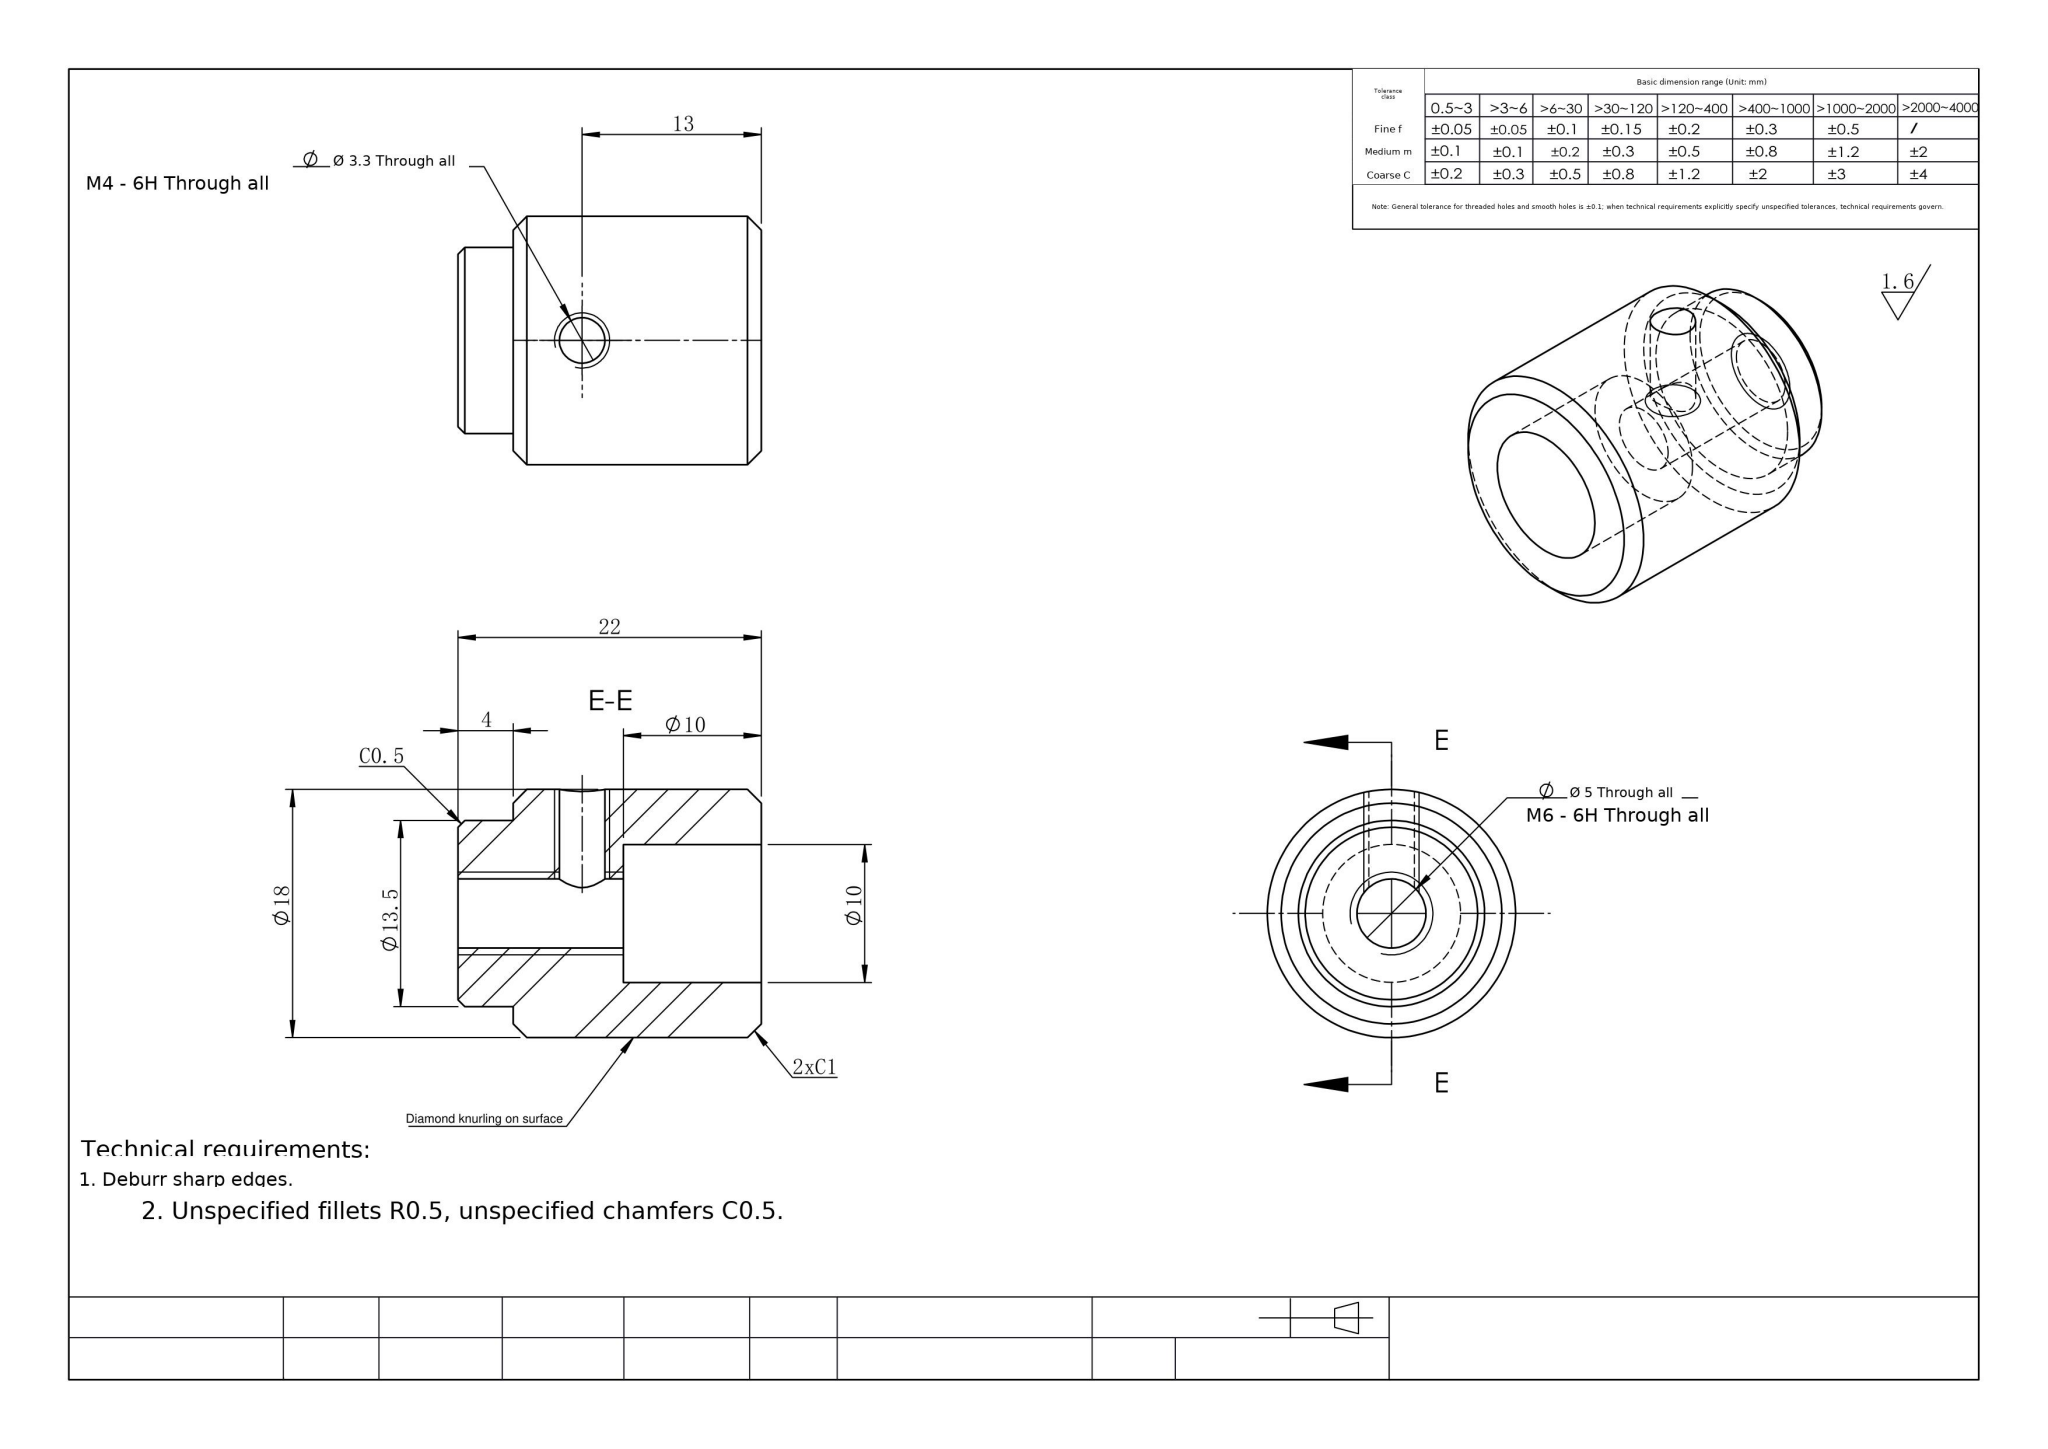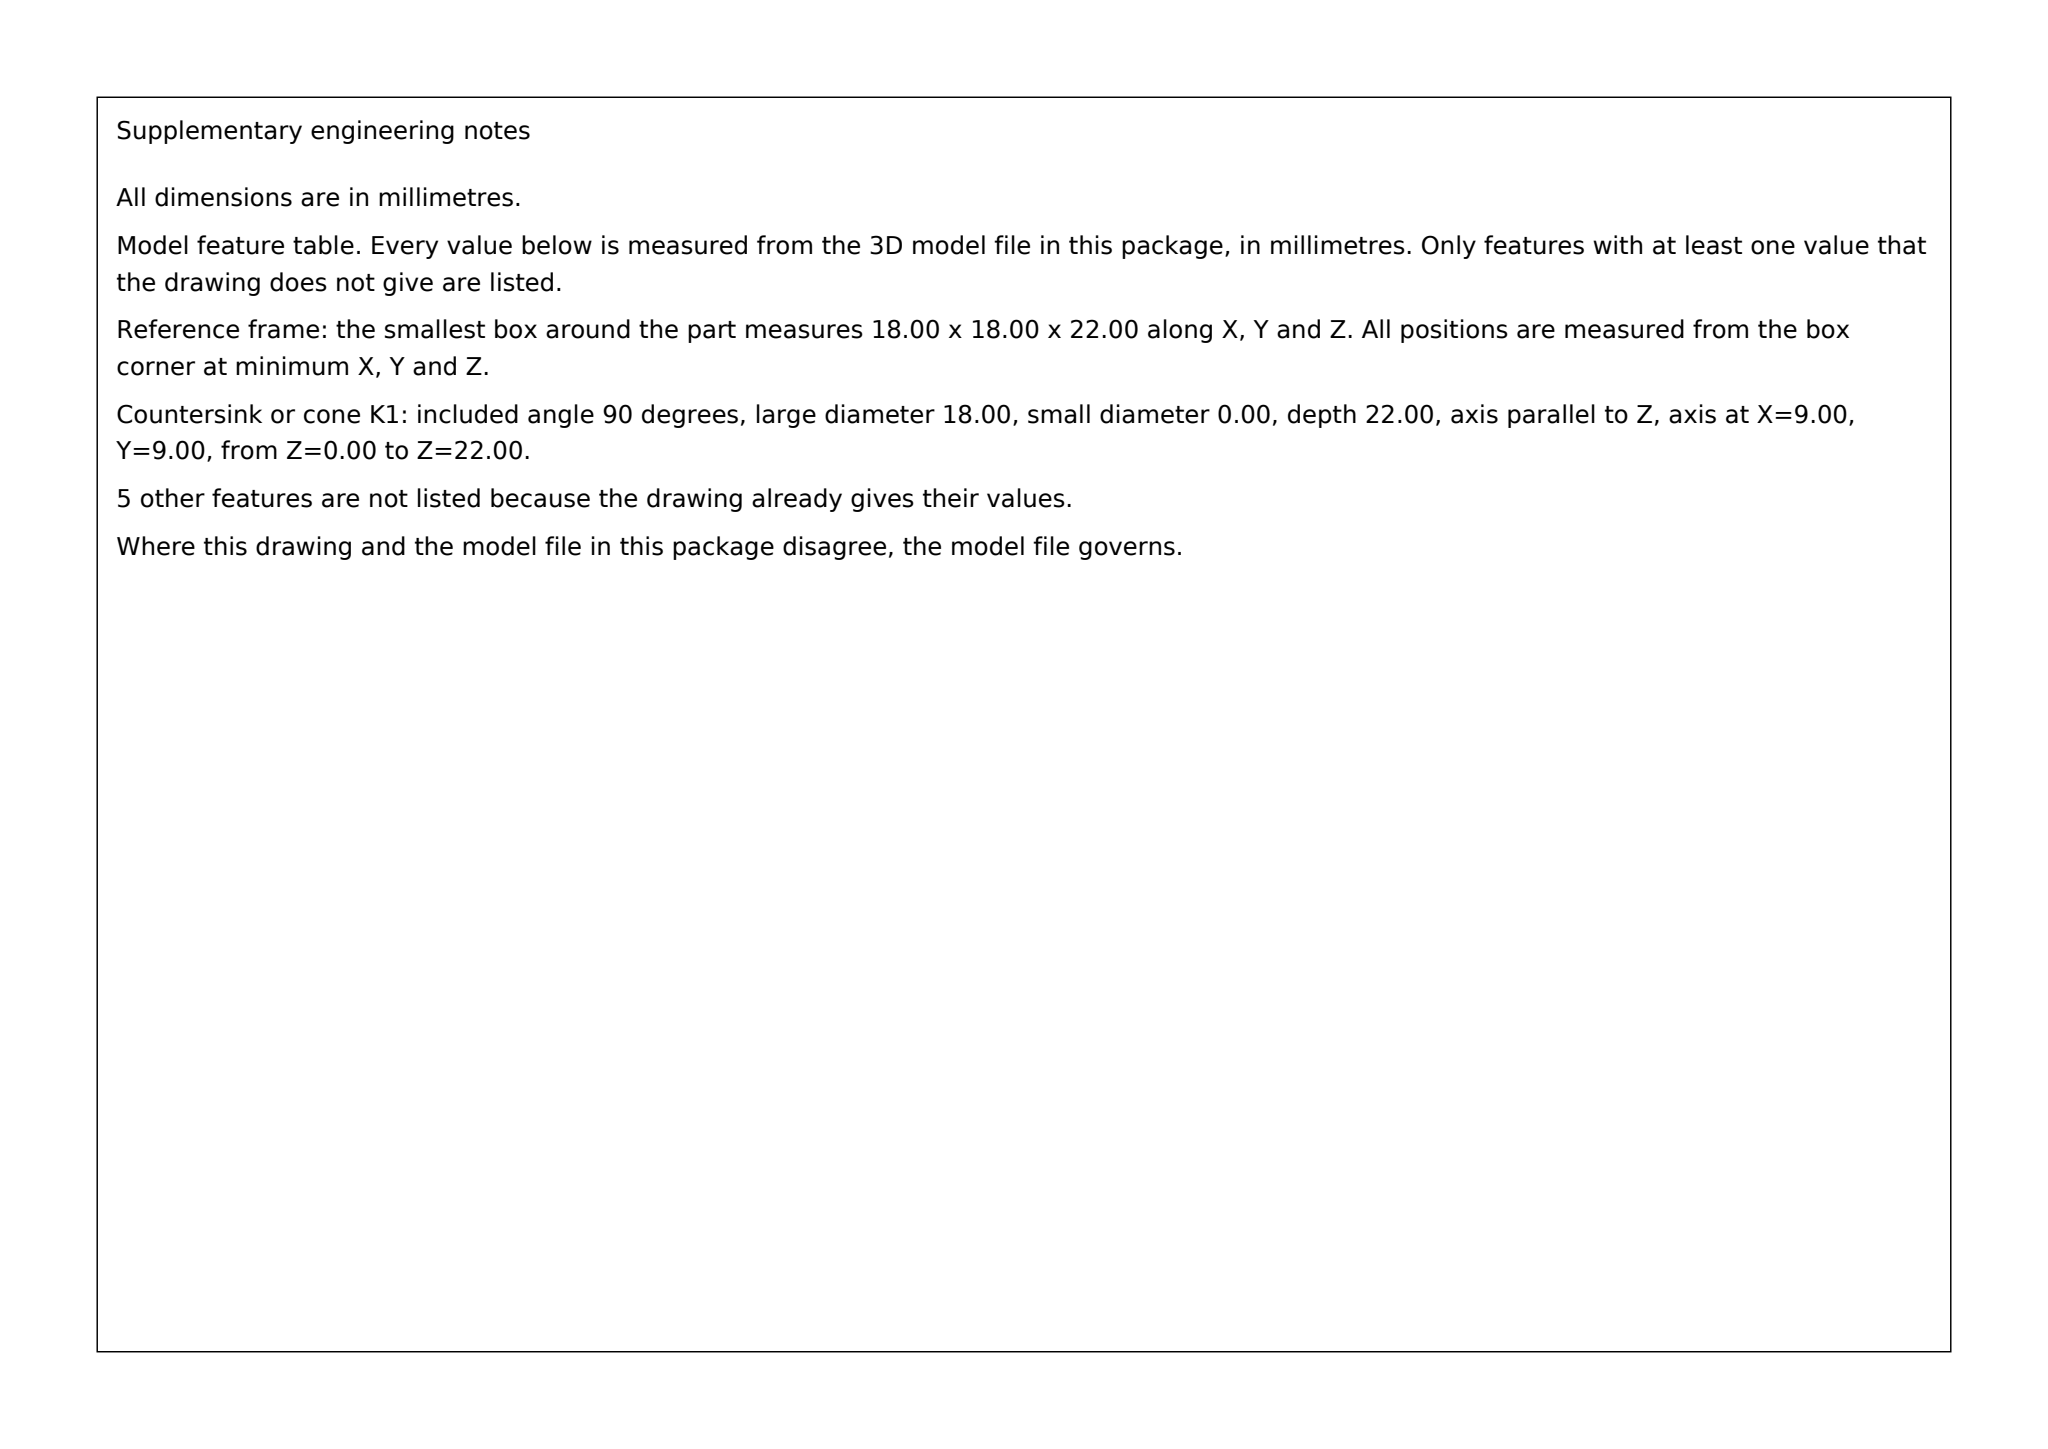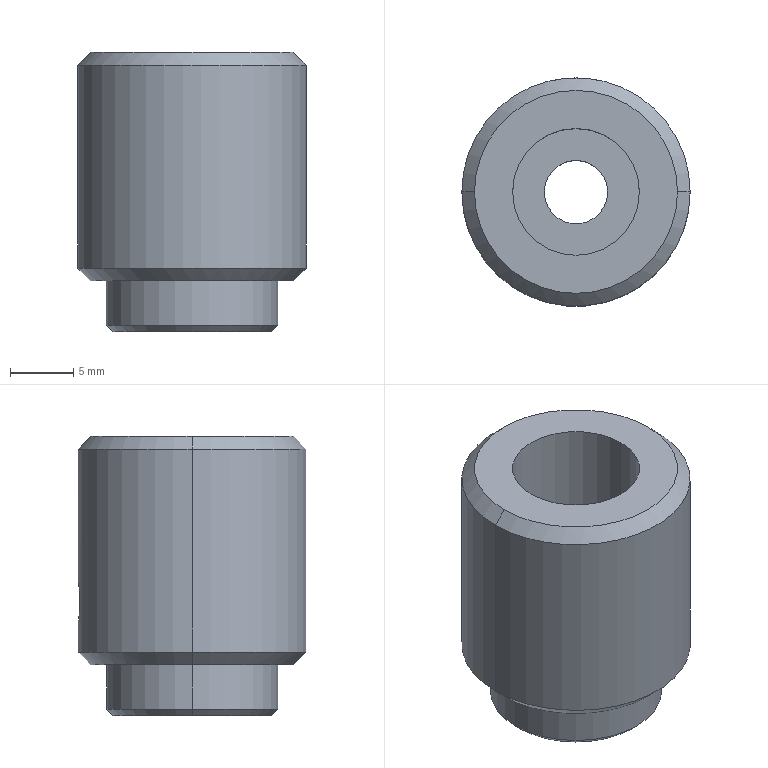Part | SolidWorks | mm | 1 solid | 20 faces | box 18 x 18 x 22 mm | volume 4016 mm3 | cylinder 10 | cone 6 | plane 4 | commonest cylinder face diameters 3.3 x2 5 x2 13.5 x2 10 x2 18 x2
build123d program:
from build123d import *

# Parameters (mm, degrees)
SKETCH1_R           = 9
BOSS_EXTRUDE1_DEPTH = 18
CHAMFER1_SIZE       = 1
SKETCH4_R           = 5
CUT_EXTRUDE1_DEPTH  = 10
SKETCH5_R           = 6.75
BOSS_EXTRUDE2_DEPTH = 4
M6_TAPPED_HOLE2_D   = 5
CHAMFER2_SIZE       = 0.5
SKETCH9_W           = 1.65
SKETCH9_H           = 9


with BuildPart() as part:
    # Sketch1 → Boss-Extrude1 (new body)
    with BuildSketch(Plane.XY):
        Circle(SKETCH1_R)
    extrude(amount=BOSS_EXTRUDE1_DEPTH)

    # Chamfer1
    chamfer1_edges = [part.edges().sort_by_distance(p)[0] for p in [
        (-9, 0, 0),
        (-9, 0, 18),
    ]]
    chamfer(chamfer1_edges, length=CHAMFER1_SIZE)

    # Sketch4 → Cut-Extrude1 (cut)
    with BuildSketch(Plane.XY.offset(18)):
        Circle(SKETCH4_R)
    extrude(amount=-CUT_EXTRUDE1_DEPTH, mode=Mode.SUBTRACT)

    # Sketch5 → Boss-Extrude2 (add)
    with BuildSketch(Plane(origin=(0, 0, 0), x_dir=(-1, 0, 0), z_dir=(0, 0, -1))):
        with Locations(Location((0, 0, 0), (0, 0, 180))):
            Circle(SKETCH5_R)
    extrude(amount=BOSS_EXTRUDE2_DEPTH)

    # M6 Tapped Hole2 (through all)
    with Locations(Plane(origin=(0, 0, -4), x_dir=(-1, 0, 0), z_dir=(0, 0, -1))):
        with Locations((0, 0)):
            Hole(M6_TAPPED_HOLE2_D / 2)

    # Chamfer2
    chamfer2_edges = [part.edges().sort_by_distance(p)[0] for p in [
        (-6.75, 0, -4),
    ]]
    chamfer(chamfer2_edges, length=CHAMFER2_SIZE)

    # Sketch9 → M4 Tapped Hole1 (revolve, cut)
    with BuildSketch(Plane(origin=(0, 0, 5), x_dir=(0, 0, -1), z_dir=(1, 0, 0))):
        with Locations((0.825, 4.5)):
            Rectangle(SKETCH9_W, SKETCH9_H)
    revolve(axis=Axis((0, -6.35, 5), (0, 1, 0)), mode=Mode.SUBTRACT)


solid = part.part
STEP:
#1=CARTESIAN_POINT('',(0.,9.,6.65));
#2=VERTEX_POINT('',#1);
#3=CARTESIAN_POINT('',(0.,9.,3.35));
#4=VERTEX_POINT('',#3);
#5=CARTESIAN_POINT('',(0.,9.,6.65));
#6=CARTESIAN_POINT('',(-0.2156,9.,6.65));
#7=CARTESIAN_POINT('',(-0.4331,8.992,6.607));
#8=CARTESIAN_POINT('',(-0.8303,8.964,6.442));
#9=CARTESIAN_POINT('',(-1.014,8.944,6.319));
#10=CARTESIAN_POINT('',(-1.242,8.914,6.091));
#11=CARTESIAN_POINT('',(-1.312,8.904,6.007));
#12=CARTESIAN_POINT('',(-1.431,8.886,5.828));
#13=CARTESIAN_POINT('',(-1.482,8.877,5.733));
#14=CARTESIAN_POINT('',(-1.607,8.856,5.433));
#15=CARTESIAN_POINT('',(-1.65,8.847,5.219));
#16=CARTESIAN_POINT('',(-1.65,8.847,4.892));
#17=CARTESIAN_POINT('',(-1.639,8.849,4.785));
#18=CARTESIAN_POINT('',(-1.598,8.857,4.573));
#19=CARTESIAN_POINT('',(-1.566,8.863,4.468));
#20=CARTESIAN_POINT('',(-1.483,8.877,4.269));
#21=CARTESIAN_POINT('',(-1.432,8.885,4.174));
#22=CARTESIAN_POINT('',(-1.313,8.904,3.994));
#23=CARTESIAN_POINT('',(-1.243,8.914,3.91));
#24=CARTESIAN_POINT('',(-1.016,8.944,3.682));
#25=CARTESIAN_POINT('',(-0.8322,8.964,3.559));
#26=CARTESIAN_POINT('',(-0.4354,8.992,3.394));
#27=CARTESIAN_POINT('',(-0.2185,9.,3.35));
#28=CARTESIAN_POINT('',(0.,9.,3.35));
#29=B_SPLINE_CURVE_WITH_KNOTS('',3,(#5,#6,#7,#8,#9,#10,#11,#12,#13,#14,#15,#16,#17,#18,#19,#20,#21,#22,#23,#24,#25,#26,#27,#28),.UNSPECIFIED.,.F.,.F.,(4,2,2,2,2,2,2,2,2,2,2,4),(0.00517,0.005816,0.006462,0.006785,0.007108,0.007754,0.008077,0.0084,0.008723,0.009046,0.009692,0.01034),.UNSPECIFIED.);
#30=EDGE_CURVE('',#2,#4,#29,.T.);
#31=ORIENTED_EDGE('',*,*,#30,.F.);
#32=CARTESIAN_POINT('',(0.,2.5,6.65));
#33=VERTEX_POINT('',#32);
#34=CARTESIAN_POINT('',(0.,0.,6.65));
#35=DIRECTION('',(0.,-1.,0.));
#36=VECTOR('',#35,1000.);
#37=LINE('',#34,#36);
#38=EDGE_CURVE('',#2,#33,#37,.T.);
#39=ORIENTED_EDGE('',*,*,#38,.T.);
#40=CARTESIAN_POINT('',(0.,2.5,3.35));
#41=VERTEX_POINT('',#40);
#42=CARTESIAN_POINT('',(0.,2.5,3.35));
#43=CARTESIAN_POINT('',(-0.1128,2.5,3.35));
#44=CARTESIAN_POINT('',(-0.2231,2.492,3.361));
#45=CARTESIAN_POINT('',(-0.4392,2.464,3.406));
#46=CARTESIAN_POINT('',(-0.5457,2.442,3.439));
#47=CARTESIAN_POINT('',(-0.8444,2.362,3.566));
#48=CARTESIAN_POINT('',(-1.022,2.287,3.688));
#49=CARTESIAN_POINT('',(-1.243,2.171,3.91));
#50=CARTESIAN_POINT('',(-1.31,2.13,3.992));
#51=CARTESIAN_POINT('',(-1.427,2.054,4.165));
#52=CARTESIAN_POINT('',(-1.477,2.017,4.257));
#53=CARTESIAN_POINT('',(-1.602,1.922,4.552));
#54=CARTESIAN_POINT('',(-1.65,1.878,4.775));
#55=CARTESIAN_POINT('',(-1.65,1.878,5.222));
#56=CARTESIAN_POINT('',(-1.604,1.921,5.443));
#57=CARTESIAN_POINT('',(-1.437,2.048,5.839));
#58=CARTESIAN_POINT('',(-1.318,2.131,6.015));
#59=CARTESIAN_POINT('',(-1.096,2.249,6.238));
#60=CARTESIAN_POINT('',(-1.015,2.287,6.305));
#61=CARTESIAN_POINT('',(-0.8408,2.356,6.424));
#62=CARTESIAN_POINT('',(-0.7457,2.388,6.476));
#63=CARTESIAN_POINT('',(-0.5456,2.442,6.561));
#64=CARTESIAN_POINT('',(-0.4413,2.463,6.594));
#65=CARTESIAN_POINT('',(-0.2236,2.492,6.639));
#66=CARTESIAN_POINT('',(-0.1111,2.5,6.65));
#67=CARTESIAN_POINT('',(0.,2.5,6.65));
#68=B_SPLINE_CURVE_WITH_KNOTS('',3,(#42,#43,#44,#45,#46,#47,#48,#49,#50,#51,#52,#53,#54,#55,#56,#57,#58,#59,#60,#61,#62,#63,#64,#65,#66,#67),.UNSPECIFIED.,.F.,.F.,(4,2,2,2,2,2,2,2,2,2,2,2,4),(0.,0.000333,0.000666,0.001332,0.001665,0.001998,0.002664,0.00333,0.003996,0.004329,0.004662,0.004995,0.005328),.UNSPECIFIED.);
#69=EDGE_CURVE('',#41,#33,#68,.T.);
#70=ORIENTED_EDGE('',*,*,#69,.F.);
#71=CARTESIAN_POINT('',(0.,0.,3.35));
#72=DIRECTION('',(0.,-1.,0.));
#73=VECTOR('',#72,1000.);
#74=LINE('',#71,#73);
#75=EDGE_CURVE('',#4,#41,#74,.T.);
#76=ORIENTED_EDGE('',*,*,#75,.F.);
#77=EDGE_LOOP('',(#31,#39,#70,#76));
#78=FACE_OUTER_BOUND('',#77,.T.);
#79=CARTESIAN_POINT('',(0.,0.,5.));
#80=DIRECTION('',(0.,-1.,0.));
#81=DIRECTION('',(0.,0.,-1.));
#82=AXIS2_PLACEMENT_3D('',#79,#80,#81);
#83=CYLINDRICAL_SURFACE('',#82,1.65);
#84=ADVANCED_FACE('',(#78),#83,.F.);
#85=CARTESIAN_POINT('',(-6.25,0.,-4.));
#86=VERTEX_POINT('',#85);
#87=CARTESIAN_POINT('',(6.25,0.,-4.));
#88=VERTEX_POINT('',#87);
#89=CARTESIAN_POINT('',(0.,0.,-4.));
#90=DIRECTION('',(0.,0.,-1.));
#91=DIRECTION('',(-1.,0.,0.));
#92=AXIS2_PLACEMENT_3D('',#89,#90,#91);
#93=CIRCLE('',#92,6.25);
#94=EDGE_CURVE('',#86,#88,#93,.T.);
#95=ORIENTED_EDGE('',*,*,#94,.F.);
#96=CARTESIAN_POINT('',(-6.75,0.,-3.5));
#97=VERTEX_POINT('',#96);
#98=CARTESIAN_POINT('',(-6.25,0.,-4.));
#99=DIRECTION('',(-0.7071,0.,0.7071));
#100=VECTOR('',#99,1000.);
#101=LINE('',#98,#100);
#102=EDGE_CURVE('',#86,#97,#101,.T.);
#103=ORIENTED_EDGE('',*,*,#102,.T.);
#104=CARTESIAN_POINT('',(6.75,0.,-3.5));
#105=VERTEX_POINT('',#104);
#106=CARTESIAN_POINT('',(0.,0.,-3.5));
#107=DIRECTION('',(0.,0.,1.));
#108=DIRECTION('',(-1.,0.,0.));
#109=AXIS2_PLACEMENT_3D('',#106,#107,#108);
#110=CIRCLE('',#109,6.75);
#111=EDGE_CURVE('',#105,#97,#110,.T.);
#112=ORIENTED_EDGE('',*,*,#111,.F.);
#113=CARTESIAN_POINT('',(6.25,0.,-4.));
#114=DIRECTION('',(0.7071,0.,0.7071));
#115=VECTOR('',#114,1000.);
#116=LINE('',#113,#115);
#117=EDGE_CURVE('',#88,#105,#116,.T.);
#118=ORIENTED_EDGE('',*,*,#117,.F.);
#119=EDGE_LOOP('',(#95,#103,#112,#118));
#120=FACE_OUTER_BOUND('',#119,.T.);
#121=CARTESIAN_POINT('',(0.,0.,-4.));
#122=DIRECTION('',(0.,0.,1.));
#123=DIRECTION('',(1.,0.,0.));
#124=AXIS2_PLACEMENT_3D('',#121,#122,#123);
#125=CONICAL_SURFACE('',#124,6.25,0.7854);
#126=ADVANCED_FACE('',(#120),#125,.T.);
#127=CARTESIAN_POINT('',(-2.5,0.,8.));
#128=VERTEX_POINT('',#127);
#129=CARTESIAN_POINT('',(2.5,0.,8.));
#130=VERTEX_POINT('',#129);
#131=CARTESIAN_POINT('',(0.,0.,8.));
#132=DIRECTION('',(0.,0.,1.));
#133=DIRECTION('',(1.,0.,0.));
#134=AXIS2_PLACEMENT_3D('',#131,#132,#133);
#135=CIRCLE('',#134,2.5);
#136=EDGE_CURVE('',#128,#130,#135,.T.);
#137=ORIENTED_EDGE('',*,*,#136,.T.);
#138=CARTESIAN_POINT('',(2.5,0.,-4.));
#139=VERTEX_POINT('',#138);
#140=CARTESIAN_POINT('',(2.5,0.,-4.));
#141=DIRECTION('',(0.,0.,-1.));
#142=VECTOR('',#141,1000.);
#143=LINE('',#140,#142);
#144=EDGE_CURVE('',#130,#139,#143,.T.);
#145=ORIENTED_EDGE('',*,*,#144,.T.);
#146=CARTESIAN_POINT('',(-2.5,0.,-4.));
#147=VERTEX_POINT('',#146);
#148=CARTESIAN_POINT('',(0.,0.,-4.));
#149=DIRECTION('',(0.,0.,-1.));
#150=DIRECTION('',(-1.,0.,0.));
#151=AXIS2_PLACEMENT_3D('',#148,#149,#150);
#152=CIRCLE('',#151,2.5);
#153=EDGE_CURVE('',#139,#147,#152,.T.);
#154=ORIENTED_EDGE('',*,*,#153,.T.);
#155=CARTESIAN_POINT('',(-2.5,0.,-4.));
#156=DIRECTION('',(0.,0.,-1.));
#157=VECTOR('',#156,1000.);
#158=LINE('',#155,#157);
#159=EDGE_CURVE('',#128,#147,#158,.T.);
#160=ORIENTED_EDGE('',*,*,#159,.F.);
#161=EDGE_LOOP('',(#137,#145,#154,#160));
#162=FACE_OUTER_BOUND('',#161,.T.);
#163=CARTESIAN_POINT('',(0.,0.,-4.));
#164=DIRECTION('',(0.,0.,-1.));
#165=DIRECTION('',(-1.,0.,0.));
#166=AXIS2_PLACEMENT_3D('',#163,#164,#165);
#167=CYLINDRICAL_SURFACE('',#166,2.5);
#168=ADVANCED_FACE('',(#162),#167,.F.);
#169=ORIENTED_EDGE('',*,*,#111,.T.);
#170=CARTESIAN_POINT('',(-6.75,0.,0.));
#171=VERTEX_POINT('',#170);
#172=CARTESIAN_POINT('',(-6.75,0.,-4.));
#173=DIRECTION('',(0.,0.,1.));
#174=VECTOR('',#173,1000.);
#175=LINE('',#172,#174);
#176=EDGE_CURVE('',#97,#171,#175,.T.);
#177=ORIENTED_EDGE('',*,*,#176,.T.);
#178=CARTESIAN_POINT('',(6.75,0.,0.));
#179=VERTEX_POINT('',#178);
#180=CARTESIAN_POINT('',(0.,0.,0.));
#181=DIRECTION('',(0.,0.,-1.));
#182=DIRECTION('',(1.,0.,0.));
#183=AXIS2_PLACEMENT_3D('',#180,#181,#182);
#184=CIRCLE('',#183,6.75);
#185=EDGE_CURVE('',#171,#179,#184,.T.);
#186=ORIENTED_EDGE('',*,*,#185,.T.);
#187=CARTESIAN_POINT('',(6.75,0.,-4.));
#188=DIRECTION('',(0.,0.,1.));
#189=VECTOR('',#188,1000.);
#190=LINE('',#187,#189);
#191=EDGE_CURVE('',#105,#179,#190,.T.);
#192=ORIENTED_EDGE('',*,*,#191,.F.);
#193=EDGE_LOOP('',(#169,#177,#186,#192));
#194=FACE_OUTER_BOUND('',#193,.T.);
#195=CARTESIAN_POINT('',(0.,0.,-4.));
#196=DIRECTION('',(0.,0.,1.));
#197=DIRECTION('',(1.,0.,0.));
#198=AXIS2_PLACEMENT_3D('',#195,#196,#197);
#199=CYLINDRICAL_SURFACE('',#198,6.75);
#200=ADVANCED_FACE('',(#194),#199,.T.);
#201=CARTESIAN_POINT('',(-5.,0.,8.));
#202=VERTEX_POINT('',#201);
#203=CARTESIAN_POINT('',(5.,0.,8.));
#204=VERTEX_POINT('',#203);
#205=CARTESIAN_POINT('',(0.,0.,8.));
#206=DIRECTION('',(0.,0.,1.));
#207=DIRECTION('',(1.,0.,0.));
#208=AXIS2_PLACEMENT_3D('',#205,#206,#207);
#209=CIRCLE('',#208,5.);
#210=EDGE_CURVE('',#202,#204,#209,.T.);
#211=ORIENTED_EDGE('',*,*,#210,.F.);
#212=CARTESIAN_POINT('',(-5.,0.,18.));
#213=VERTEX_POINT('',#212);
#214=CARTESIAN_POINT('',(-5.,0.,8.));
#215=DIRECTION('',(0.,0.,1.));
#216=VECTOR('',#215,1000.);
#217=LINE('',#214,#216);
#218=EDGE_CURVE('',#202,#213,#217,.T.);
#219=ORIENTED_EDGE('',*,*,#218,.T.);
#220=CARTESIAN_POINT('',(5.,0.,18.));
#221=VERTEX_POINT('',#220);
#222=CARTESIAN_POINT('',(0.,0.,18.));
#223=DIRECTION('',(0.,0.,1.));
#224=DIRECTION('',(1.,0.,0.));
#225=AXIS2_PLACEMENT_3D('',#222,#223,#224);
#226=CIRCLE('',#225,5.);
#227=EDGE_CURVE('',#213,#221,#226,.T.);
#228=ORIENTED_EDGE('',*,*,#227,.T.);
#229=CARTESIAN_POINT('',(5.,0.,8.));
#230=DIRECTION('',(0.,0.,1.));
#231=VECTOR('',#230,1000.);
#232=LINE('',#229,#231);
#233=EDGE_CURVE('',#204,#221,#232,.T.);
#234=ORIENTED_EDGE('',*,*,#233,.F.);
#235=EDGE_LOOP('',(#211,#219,#228,#234));
#236=FACE_OUTER_BOUND('',#235,.T.);
#237=CARTESIAN_POINT('',(0.,0.,8.));
#238=DIRECTION('',(0.,0.,1.));
#239=DIRECTION('',(1.,0.,0.));
#240=AXIS2_PLACEMENT_3D('',#237,#238,#239);
#241=CYLINDRICAL_SURFACE('',#240,5.);
#242=ADVANCED_FACE('',(#236),#241,.F.);
#243=CARTESIAN_POINT('',(-8.,0.,0.));
#244=VERTEX_POINT('',#243);
#245=CARTESIAN_POINT('',(8.,0.,0.));
#246=VERTEX_POINT('',#245);
#247=CARTESIAN_POINT('',(0.,0.,0.));
#248=DIRECTION('',(0.,0.,-1.));
#249=DIRECTION('',(1.,0.,0.));
#250=AXIS2_PLACEMENT_3D('',#247,#248,#249);
#251=CIRCLE('',#250,8.);
#252=EDGE_CURVE('',#244,#246,#251,.T.);
#253=ORIENTED_EDGE('',*,*,#252,.F.);
#254=CARTESIAN_POINT('',(-9.,0.,1.));
#255=VERTEX_POINT('',#254);
#256=CARTESIAN_POINT('',(-9.,0.,1.));
#257=DIRECTION('',(-0.7071,0.,0.7071));
#258=VECTOR('',#257,1000.);
#259=LINE('',#256,#258);
#260=EDGE_CURVE('',#244,#255,#259,.T.);
#261=ORIENTED_EDGE('',*,*,#260,.T.);
#262=CARTESIAN_POINT('',(9.,0.,1.));
#263=VERTEX_POINT('',#262);
#264=CARTESIAN_POINT('',(0.,0.,1.));
#265=DIRECTION('',(0.,0.,1.));
#266=DIRECTION('',(1.,0.,0.));
#267=AXIS2_PLACEMENT_3D('',#264,#265,#266);
#268=CIRCLE('',#267,9.);
#269=EDGE_CURVE('',#263,#255,#268,.T.);
#270=ORIENTED_EDGE('',*,*,#269,.F.);
#271=CARTESIAN_POINT('',(9.,0.,1.));
#272=DIRECTION('',(0.7071,0.,0.7071));
#273=VECTOR('',#272,1000.);
#274=LINE('',#271,#273);
#275=EDGE_CURVE('',#246,#263,#274,.T.);
#276=ORIENTED_EDGE('',*,*,#275,.F.);
#277=EDGE_LOOP('',(#253,#261,#270,#276));
#278=FACE_OUTER_BOUND('',#277,.T.);
#279=CARTESIAN_POINT('',(0.,0.,1.));
#280=DIRECTION('',(0.,0.,1.));
#281=DIRECTION('',(1.,0.,0.));
#282=AXIS2_PLACEMENT_3D('',#279,#280,#281);
#283=CONICAL_SURFACE('',#282,9.,0.7854);
#284=ADVANCED_FACE('',(#278),#283,.T.);
#285=CARTESIAN_POINT('',(8.,0.,18.));
#286=VERTEX_POINT('',#285);
#287=CARTESIAN_POINT('',(-8.,0.,18.));
#288=VERTEX_POINT('',#287);
#289=CARTESIAN_POINT('',(0.,0.,18.));
#290=DIRECTION('',(0.,0.,1.));
#291=DIRECTION('',(1.,0.,0.));
#292=AXIS2_PLACEMENT_3D('',#289,#290,#291);
#293=CIRCLE('',#292,8.);
#294=EDGE_CURVE('',#286,#288,#293,.T.);
#295=ORIENTED_EDGE('',*,*,#294,.F.);
#296=CARTESIAN_POINT('',(9.,0.,17.));
#297=VERTEX_POINT('',#296);
#298=CARTESIAN_POINT('',(8.,0.,18.));
#299=DIRECTION('',(0.7071,0.,-0.7071));
#300=VECTOR('',#299,1000.);
#301=LINE('',#298,#300);
#302=EDGE_CURVE('',#286,#297,#301,.T.);
#303=ORIENTED_EDGE('',*,*,#302,.T.);
#304=CARTESIAN_POINT('',(-9.,0.,17.));
#305=VERTEX_POINT('',#304);
#306=CARTESIAN_POINT('',(0.,0.,17.));
#307=DIRECTION('',(0.,0.,-1.));
#308=DIRECTION('',(1.,0.,0.));
#309=AXIS2_PLACEMENT_3D('',#306,#307,#308);
#310=CIRCLE('',#309,9.);
#311=EDGE_CURVE('',#305,#297,#310,.T.);
#312=ORIENTED_EDGE('',*,*,#311,.F.);
#313=CARTESIAN_POINT('',(-8.,0.,18.));
#314=DIRECTION('',(-0.7071,0.,-0.7071));
#315=VECTOR('',#314,1000.);
#316=LINE('',#313,#315);
#317=EDGE_CURVE('',#288,#305,#316,.T.);
#318=ORIENTED_EDGE('',*,*,#317,.F.);
#319=EDGE_LOOP('',(#295,#303,#312,#318));
#320=FACE_OUTER_BOUND('',#319,.T.);
#321=CARTESIAN_POINT('',(0.,0.,18.));
#322=DIRECTION('',(0.,0.,-1.));
#323=DIRECTION('',(-1.,0.,0.));
#324=AXIS2_PLACEMENT_3D('',#321,#322,#323);
#325=CONICAL_SURFACE('',#324,8.,0.7854);
#326=ADVANCED_FACE('',(#320),#325,.T.);
#327=CARTESIAN_POINT('',(0.,9.,3.35));
#328=CARTESIAN_POINT('',(0.1093,9.,3.35));
#329=CARTESIAN_POINT('',(0.2167,8.998,3.361));
#330=CARTESIAN_POINT('',(0.4279,8.99,3.403));
#331=CARTESIAN_POINT('',(0.5328,8.985,3.435));
#332=CARTESIAN_POINT('',(0.7325,8.971,3.518));
#333=CARTESIAN_POINT('',(0.8272,8.962,3.568));
#334=CARTESIAN_POINT('',(1.006,8.944,3.688));
#335=CARTESIAN_POINT('',(1.091,8.934,3.758));
#336=CARTESIAN_POINT('',(1.319,8.904,3.985));
#337=CARTESIAN_POINT('',(1.442,8.884,4.169));
#338=CARTESIAN_POINT('',(1.606,8.856,4.566));
#339=CARTESIAN_POINT('',(1.65,8.847,4.784));
#340=CARTESIAN_POINT('',(1.65,8.847,5.107));
#341=CARTESIAN_POINT('',(1.639,8.849,5.217));
#342=CARTESIAN_POINT('',(1.597,8.857,5.429));
#343=CARTESIAN_POINT('',(1.566,8.863,5.532));
#344=CARTESIAN_POINT('',(1.441,8.884,5.832));
#345=CARTESIAN_POINT('',(1.32,8.904,6.013));
#346=CARTESIAN_POINT('',(1.09,8.934,6.244));
#347=CARTESIAN_POINT('',(1.007,8.944,6.312));
#348=CARTESIAN_POINT('',(0.8283,8.962,6.431));
#349=CARTESIAN_POINT('',(0.7317,8.971,6.483));
#350=CARTESIAN_POINT('',(0.5322,8.985,6.566));
#351=CARTESIAN_POINT('',(0.4293,8.99,6.597));
#352=CARTESIAN_POINT('',(0.2173,8.998,6.639));
#353=CARTESIAN_POINT('',(0.1078,9.,6.65));
#354=CARTESIAN_POINT('',(0.,9.,6.65));
#355=B_SPLINE_CURVE_WITH_KNOTS('',3,(#327,#328,#329,#330,#331,#332,#333,#334,#335,#336,#337,#338,#339,#340,#341,#342,#343,#344,#345,#346,#347,#348,#349,#350,#351,#352,#353,#354),.UNSPECIFIED.,.F.,.F.,(4,2,2,2,2,2,2,2,2,2,2,2,2,4),(0.,0.0003231,0.0006462,0.0009693,0.001292,0.001939,0.002585,0.002908,0.003231,0.003877,0.0042,0.004523,0.004846,0.00517),.UNSPECIFIED.);
#356=EDGE_CURVE('',#4,#2,#355,.T.);
#357=ORIENTED_EDGE('',*,*,#356,.T.);
#358=ORIENTED_EDGE('',*,*,#30,.T.);
#359=EDGE_LOOP('',(#357,#358));
#360=FACE_BOUND('',#359,.T.);
#361=ORIENTED_EDGE('',*,*,#311,.T.);
#362=CARTESIAN_POINT('',(9.,0.,18.));
#363=DIRECTION('',(0.,0.,-1.));
#364=VECTOR('',#363,1000.);
#365=LINE('',#362,#364);
#366=EDGE_CURVE('',#297,#263,#365,.T.);
#367=ORIENTED_EDGE('',*,*,#366,.T.);
#368=ORIENTED_EDGE('',*,*,#269,.T.);
#369=CARTESIAN_POINT('',(-9.,0.,18.));
#370=DIRECTION('',(0.,0.,-1.));
#371=VECTOR('',#370,1000.);
#372=LINE('',#369,#371);
#373=EDGE_CURVE('',#305,#255,#372,.T.);
#374=ORIENTED_EDGE('',*,*,#373,.F.);
#375=EDGE_LOOP('',(#361,#367,#368,#374));
#376=FACE_OUTER_BOUND('',#375,.T.);
#377=CARTESIAN_POINT('',(0.,0.,18.));
#378=DIRECTION('',(0.,0.,-1.));
#379=DIRECTION('',(-1.,0.,0.));
#380=AXIS2_PLACEMENT_3D('',#377,#378,#379);
#381=CYLINDRICAL_SURFACE('',#380,9.);
#382=ADVANCED_FACE('',(#360,#376),#381,.T.);
#383=ORIENTED_EDGE('',*,*,#366,.F.);
#384=CARTESIAN_POINT('',(0.,0.,17.));
#385=DIRECTION('',(0.,0.,-1.));
#386=DIRECTION('',(1.,0.,0.));
#387=AXIS2_PLACEMENT_3D('',#384,#385,#386);
#388=CIRCLE('',#387,9.);
#389=EDGE_CURVE('',#297,#305,#388,.T.);
#390=ORIENTED_EDGE('',*,*,#389,.T.);
#391=ORIENTED_EDGE('',*,*,#373,.T.);
#392=CARTESIAN_POINT('',(0.,0.,1.));
#393=DIRECTION('',(0.,0.,1.));
#394=DIRECTION('',(1.,0.,0.));
#395=AXIS2_PLACEMENT_3D('',#392,#393,#394);
#396=CIRCLE('',#395,9.);
#397=EDGE_CURVE('',#255,#263,#396,.T.);
#398=ORIENTED_EDGE('',*,*,#397,.T.);
#399=EDGE_LOOP('',(#383,#390,#391,#398));
#400=FACE_OUTER_BOUND('',#399,.T.);
#401=CARTESIAN_POINT('',(0.,0.,18.));
#402=DIRECTION('',(0.,0.,-1.));
#403=DIRECTION('',(-1.,0.,0.));
#404=AXIS2_PLACEMENT_3D('',#401,#402,#403);
#405=CYLINDRICAL_SURFACE('',#404,9.);
#406=ADVANCED_FACE('',(#400),#405,.T.);
#407=CARTESIAN_POINT('',(0.,0.,18.));
#408=DIRECTION('',(0.,0.,1.));
#409=DIRECTION('',(1.,0.,0.));
#410=AXIS2_PLACEMENT_3D('',#407,#408,#409);
#411=CIRCLE('',#410,5.);
#412=EDGE_CURVE('',#221,#213,#411,.T.);
#413=ORIENTED_EDGE('',*,*,#412,.F.);
#414=ORIENTED_EDGE('',*,*,#227,.F.);
#415=EDGE_LOOP('',(#413,#414));
#416=FACE_BOUND('',#415,.T.);
#417=CARTESIAN_POINT('',(0.,0.,18.));
#418=DIRECTION('',(0.,0.,1.));
#419=DIRECTION('',(1.,0.,0.));
#420=AXIS2_PLACEMENT_3D('',#417,#418,#419);
#421=CIRCLE('',#420,8.);
#422=EDGE_CURVE('',#288,#286,#421,.T.);
#423=ORIENTED_EDGE('',*,*,#422,.T.);
#424=ORIENTED_EDGE('',*,*,#294,.T.);
#425=EDGE_LOOP('',(#423,#424));
#426=FACE_OUTER_BOUND('',#425,.T.);
#427=CARTESIAN_POINT('',(0.,0.,18.));
#428=DIRECTION('',(0.,0.,1.));
#429=DIRECTION('',(1.,0.,0.));
#430=AXIS2_PLACEMENT_3D('',#427,#428,#429);
#431=PLANE('',#430);
#432=ADVANCED_FACE('',(#416,#426),#431,.T.);
#433=CARTESIAN_POINT('',(0.,0.,0.));
#434=DIRECTION('',(0.,0.,-1.));
#435=DIRECTION('',(1.,0.,0.));
#436=AXIS2_PLACEMENT_3D('',#433,#434,#435);
#437=CIRCLE('',#436,6.75);
#438=EDGE_CURVE('',#179,#171,#437,.T.);
#439=ORIENTED_EDGE('',*,*,#438,.F.);
#440=ORIENTED_EDGE('',*,*,#185,.F.);
#441=EDGE_LOOP('',(#439,#440));
#442=FACE_BOUND('',#441,.T.);
#443=CARTESIAN_POINT('',(0.,0.,0.));
#444=DIRECTION('',(0.,0.,-1.));
#445=DIRECTION('',(1.,0.,0.));
#446=AXIS2_PLACEMENT_3D('',#443,#444,#445);
#447=CIRCLE('',#446,8.);
#448=EDGE_CURVE('',#246,#244,#447,.T.);
#449=ORIENTED_EDGE('',*,*,#448,.T.);
#450=ORIENTED_EDGE('',*,*,#252,.T.);
#451=EDGE_LOOP('',(#449,#450));
#452=FACE_OUTER_BOUND('',#451,.T.);
#453=CARTESIAN_POINT('',(0.,0.,0.));
#454=DIRECTION('',(0.,0.,1.));
#455=DIRECTION('',(1.,0.,0.));
#456=AXIS2_PLACEMENT_3D('',#453,#454,#455);
#457=PLANE('',#456);
#458=ADVANCED_FACE('',(#442,#452),#457,.F.);
#459=ORIENTED_EDGE('',*,*,#302,.F.);
#460=ORIENTED_EDGE('',*,*,#422,.F.);
#461=ORIENTED_EDGE('',*,*,#317,.T.);
#462=ORIENTED_EDGE('',*,*,#389,.F.);
#463=EDGE_LOOP('',(#459,#460,#461,#462));
#464=FACE_OUTER_BOUND('',#463,.T.);
#465=CARTESIAN_POINT('',(0.,0.,18.));
#466=DIRECTION('',(0.,0.,-1.));
#467=DIRECTION('',(-1.,0.,0.));
#468=AXIS2_PLACEMENT_3D('',#465,#466,#467);
#469=CONICAL_SURFACE('',#468,8.,0.7854);
#470=ADVANCED_FACE('',(#464),#469,.T.);
#471=ORIENTED_EDGE('',*,*,#260,.F.);
#472=ORIENTED_EDGE('',*,*,#448,.F.);
#473=ORIENTED_EDGE('',*,*,#275,.T.);
#474=ORIENTED_EDGE('',*,*,#397,.F.);
#475=EDGE_LOOP('',(#471,#472,#473,#474));
#476=FACE_OUTER_BOUND('',#475,.T.);
#477=CARTESIAN_POINT('',(0.,0.,1.));
#478=DIRECTION('',(0.,0.,1.));
#479=DIRECTION('',(1.,0.,0.));
#480=AXIS2_PLACEMENT_3D('',#477,#478,#479);
#481=CONICAL_SURFACE('',#480,9.,0.7854);
#482=ADVANCED_FACE('',(#476),#481,.T.);
#483=ORIENTED_EDGE('',*,*,#218,.F.);
#484=CARTESIAN_POINT('',(0.,0.,8.));
#485=DIRECTION('',(0.,0.,1.));
#486=DIRECTION('',(1.,0.,0.));
#487=AXIS2_PLACEMENT_3D('',#484,#485,#486);
#488=CIRCLE('',#487,5.);
#489=EDGE_CURVE('',#204,#202,#488,.T.);
#490=ORIENTED_EDGE('',*,*,#489,.F.);
#491=ORIENTED_EDGE('',*,*,#233,.T.);
#492=ORIENTED_EDGE('',*,*,#412,.T.);
#493=EDGE_LOOP('',(#483,#490,#491,#492));
#494=FACE_OUTER_BOUND('',#493,.T.);
#495=CARTESIAN_POINT('',(0.,0.,8.));
#496=DIRECTION('',(0.,0.,1.));
#497=DIRECTION('',(1.,0.,0.));
#498=AXIS2_PLACEMENT_3D('',#495,#496,#497);
#499=CYLINDRICAL_SURFACE('',#498,5.);
#500=ADVANCED_FACE('',(#494),#499,.F.);
#501=ORIENTED_EDGE('',*,*,#136,.F.);
#502=CARTESIAN_POINT('',(0.,0.,8.));
#503=DIRECTION('',(0.,0.,1.));
#504=DIRECTION('',(1.,0.,0.));
#505=AXIS2_PLACEMENT_3D('',#502,#503,#504);
#506=CIRCLE('',#505,2.5);
#507=EDGE_CURVE('',#130,#128,#506,.T.);
#508=ORIENTED_EDGE('',*,*,#507,.F.);
#509=EDGE_LOOP('',(#501,#508));
#510=FACE_BOUND('',#509,.T.);
#511=ORIENTED_EDGE('',*,*,#489,.T.);
#512=ORIENTED_EDGE('',*,*,#210,.T.);
#513=EDGE_LOOP('',(#511,#512));
#514=FACE_OUTER_BOUND('',#513,.T.);
#515=CARTESIAN_POINT('',(0.,0.,8.));
#516=DIRECTION('',(0.,0.,1.));
#517=DIRECTION('',(1.,0.,0.));
#518=AXIS2_PLACEMENT_3D('',#515,#516,#517);
#519=PLANE('',#518);
#520=ADVANCED_FACE('',(#510,#514),#519,.T.);
#521=ORIENTED_EDGE('',*,*,#176,.F.);
#522=CARTESIAN_POINT('',(0.,0.,-3.5));
#523=DIRECTION('',(0.,0.,1.));
#524=DIRECTION('',(-1.,0.,0.));
#525=AXIS2_PLACEMENT_3D('',#522,#523,#524);
#526=CIRCLE('',#525,6.75);
#527=EDGE_CURVE('',#97,#105,#526,.T.);
#528=ORIENTED_EDGE('',*,*,#527,.T.);
#529=ORIENTED_EDGE('',*,*,#191,.T.);
#530=ORIENTED_EDGE('',*,*,#438,.T.);
#531=EDGE_LOOP('',(#521,#528,#529,#530));
#532=FACE_OUTER_BOUND('',#531,.T.);
#533=CARTESIAN_POINT('',(0.,0.,-4.));
#534=DIRECTION('',(0.,0.,1.));
#535=DIRECTION('',(1.,0.,0.));
#536=AXIS2_PLACEMENT_3D('',#533,#534,#535);
#537=CYLINDRICAL_SURFACE('',#536,6.75);
#538=ADVANCED_FACE('',(#532),#537,.T.);
#539=CARTESIAN_POINT('',(0.,0.,-4.));
#540=DIRECTION('',(0.,0.,-1.));
#541=DIRECTION('',(-1.,0.,0.));
#542=AXIS2_PLACEMENT_3D('',#539,#540,#541);
#543=CIRCLE('',#542,6.25);
#544=EDGE_CURVE('',#88,#86,#543,.T.);
#545=ORIENTED_EDGE('',*,*,#544,.T.);
#546=ORIENTED_EDGE('',*,*,#94,.T.);
#547=EDGE_LOOP('',(#545,#546));
#548=FACE_OUTER_BOUND('',#547,.T.);
#549=CARTESIAN_POINT('',(0.,0.,-4.));
#550=DIRECTION('',(0.,0.,-1.));
#551=DIRECTION('',(-1.,0.,0.));
#552=AXIS2_PLACEMENT_3D('',#549,#550,#551);
#553=CIRCLE('',#552,2.5);
#554=EDGE_CURVE('',#147,#139,#553,.T.);
#555=ORIENTED_EDGE('',*,*,#554,.F.);
#556=ORIENTED_EDGE('',*,*,#153,.F.);
#557=EDGE_LOOP('',(#555,#556));
#558=FACE_BOUND('',#557,.T.);
#559=CARTESIAN_POINT('',(0.,0.,-4.));
#560=DIRECTION('',(0.,0.,-1.));
#561=DIRECTION('',(-1.,0.,0.));
#562=AXIS2_PLACEMENT_3D('',#559,#560,#561);
#563=PLANE('',#562);
#564=ADVANCED_FACE('',(#548,#558),#563,.T.);
#565=ORIENTED_EDGE('',*,*,#144,.F.);
#566=ORIENTED_EDGE('',*,*,#507,.T.);
#567=ORIENTED_EDGE('',*,*,#159,.T.);
#568=ORIENTED_EDGE('',*,*,#554,.T.);
#569=EDGE_LOOP('',(#565,#566,#567,#568));
#570=FACE_OUTER_BOUND('',#569,.T.);
#571=ORIENTED_EDGE('',*,*,#69,.T.);
#572=CARTESIAN_POINT('',(0.,2.5,6.65));
#573=CARTESIAN_POINT('',(0.111,2.5,6.65));
#574=CARTESIAN_POINT('',(0.2235,2.492,6.639));
#575=CARTESIAN_POINT('',(0.4408,2.463,6.594));
#576=CARTESIAN_POINT('',(0.5451,2.442,6.561));
#577=CARTESIAN_POINT('',(0.8462,2.362,6.433));
#578=CARTESIAN_POINT('',(1.024,2.287,6.311));
#579=CARTESIAN_POINT('',(1.245,2.17,6.088));
#580=CARTESIAN_POINT('',(1.311,2.13,6.008));
#581=CARTESIAN_POINT('',(1.428,2.053,5.834));
#582=CARTESIAN_POINT('',(1.479,2.016,5.74));
#583=CARTESIAN_POINT('',(1.603,1.921,5.445));
#584=CARTESIAN_POINT('',(1.65,1.878,5.224));
#585=CARTESIAN_POINT('',(1.65,1.878,4.775));
#586=CARTESIAN_POINT('',(1.602,1.922,4.553));
#587=CARTESIAN_POINT('',(1.436,2.049,4.16));
#588=CARTESIAN_POINT('',(1.316,2.132,3.984));
#589=CARTESIAN_POINT('',(1.022,2.288,3.688));
#590=CARTESIAN_POINT('',(0.8442,2.362,3.566));
#591=CARTESIAN_POINT('',(0.5472,2.442,3.44));
#592=CARTESIAN_POINT('',(0.4407,2.463,3.406));
#593=CARTESIAN_POINT('',(0.2236,2.492,3.361));
#594=CARTESIAN_POINT('',(0.1126,2.5,3.35));
#595=CARTESIAN_POINT('',(0.,2.5,3.35));
#596=B_SPLINE_CURVE_WITH_KNOTS('',3,(#572,#573,#574,#575,#576,#577,#578,#579,#580,#581,#582,#583,#584,#585,#586,#587,#588,#589,#590,#591,#592,#593,#594,#595),.UNSPECIFIED.,.F.,.F.,(4,2,2,2,2,2,2,2,2,2,2,4),(0.005328,0.005661,0.005993,0.006658,0.006991,0.007324,0.007989,0.008654,0.009319,0.009984,0.01032,0.01065),.UNSPECIFIED.);
#597=EDGE_CURVE('',#33,#41,#596,.T.);
#598=ORIENTED_EDGE('',*,*,#597,.T.);
#599=EDGE_LOOP('',(#571,#598));
#600=FACE_BOUND('',#599,.T.);
#601=CARTESIAN_POINT('',(0.,0.,-4.));
#602=DIRECTION('',(0.,0.,-1.));
#603=DIRECTION('',(-1.,0.,0.));
#604=AXIS2_PLACEMENT_3D('',#601,#602,#603);
#605=CYLINDRICAL_SURFACE('',#604,2.5);
#606=ADVANCED_FACE('',(#570,#600),#605,.F.);
#607=ORIENTED_EDGE('',*,*,#102,.F.);
#608=ORIENTED_EDGE('',*,*,#544,.F.);
#609=ORIENTED_EDGE('',*,*,#117,.T.);
#610=ORIENTED_EDGE('',*,*,#527,.F.);
#611=EDGE_LOOP('',(#607,#608,#609,#610));
#612=FACE_OUTER_BOUND('',#611,.T.);
#613=CARTESIAN_POINT('',(0.,0.,-4.));
#614=DIRECTION('',(0.,0.,1.));
#615=DIRECTION('',(1.,0.,0.));
#616=AXIS2_PLACEMENT_3D('',#613,#614,#615);
#617=CONICAL_SURFACE('',#616,6.25,0.7854);
#618=ADVANCED_FACE('',(#612),#617,.T.);
#619=ORIENTED_EDGE('',*,*,#38,.F.);
#620=ORIENTED_EDGE('',*,*,#356,.F.);
#621=ORIENTED_EDGE('',*,*,#75,.T.);
#622=ORIENTED_EDGE('',*,*,#597,.F.);
#623=EDGE_LOOP('',(#619,#620,#621,#622));
#624=FACE_OUTER_BOUND('',#623,.T.);
#625=CARTESIAN_POINT('',(0.,0.,5.));
#626=DIRECTION('',(0.,-1.,0.));
#627=DIRECTION('',(0.,0.,-1.));
#628=AXIS2_PLACEMENT_3D('',#625,#626,#627);
#629=CYLINDRICAL_SURFACE('',#628,1.65);
#630=ADVANCED_FACE('',(#624),#629,.F.);
#631=CLOSED_SHELL('',(#84,#126,#168,#200,#242,#284,#326,#382,#406,#432,#458,#470,#482,#500,#520,#538,#564,#606,#618,#630));
#632=MANIFOLD_SOLID_BREP('',#631);
#633=CARTESIAN_POINT('',(0.,0.,0.));
#634=DIRECTION('',(0.,0.,1.));
#635=DIRECTION('',(1.,0.,0.));
#636=AXIS2_PLACEMENT_3D('',#633,#634,#635);
#637=(LENGTH_UNIT()NAMED_UNIT(*)SI_UNIT(.MILLI.,.METRE.));
#638=UNCERTAINTY_MEASURE_WITH_UNIT(LENGTH_MEASURE(0.00001),#637,'','');
#639=(NAMED_UNIT(*)PLANE_ANGLE_UNIT()SI_UNIT($,.RADIAN.));
#640=(NAMED_UNIT(*)SI_UNIT($,.STERADIAN.)SOLID_ANGLE_UNIT());
#641=(GEOMETRIC_REPRESENTATION_CONTEXT(3)GLOBAL_UNCERTAINTY_ASSIGNED_CONTEXT((#638))GLOBAL_UNIT_ASSIGNED_CONTEXT((#637,#639,#640))REPRESENTATION_CONTEXT('',''));
#642=ADVANCED_BREP_SHAPE_REPRESENTATION('',(#632,#636),#641);